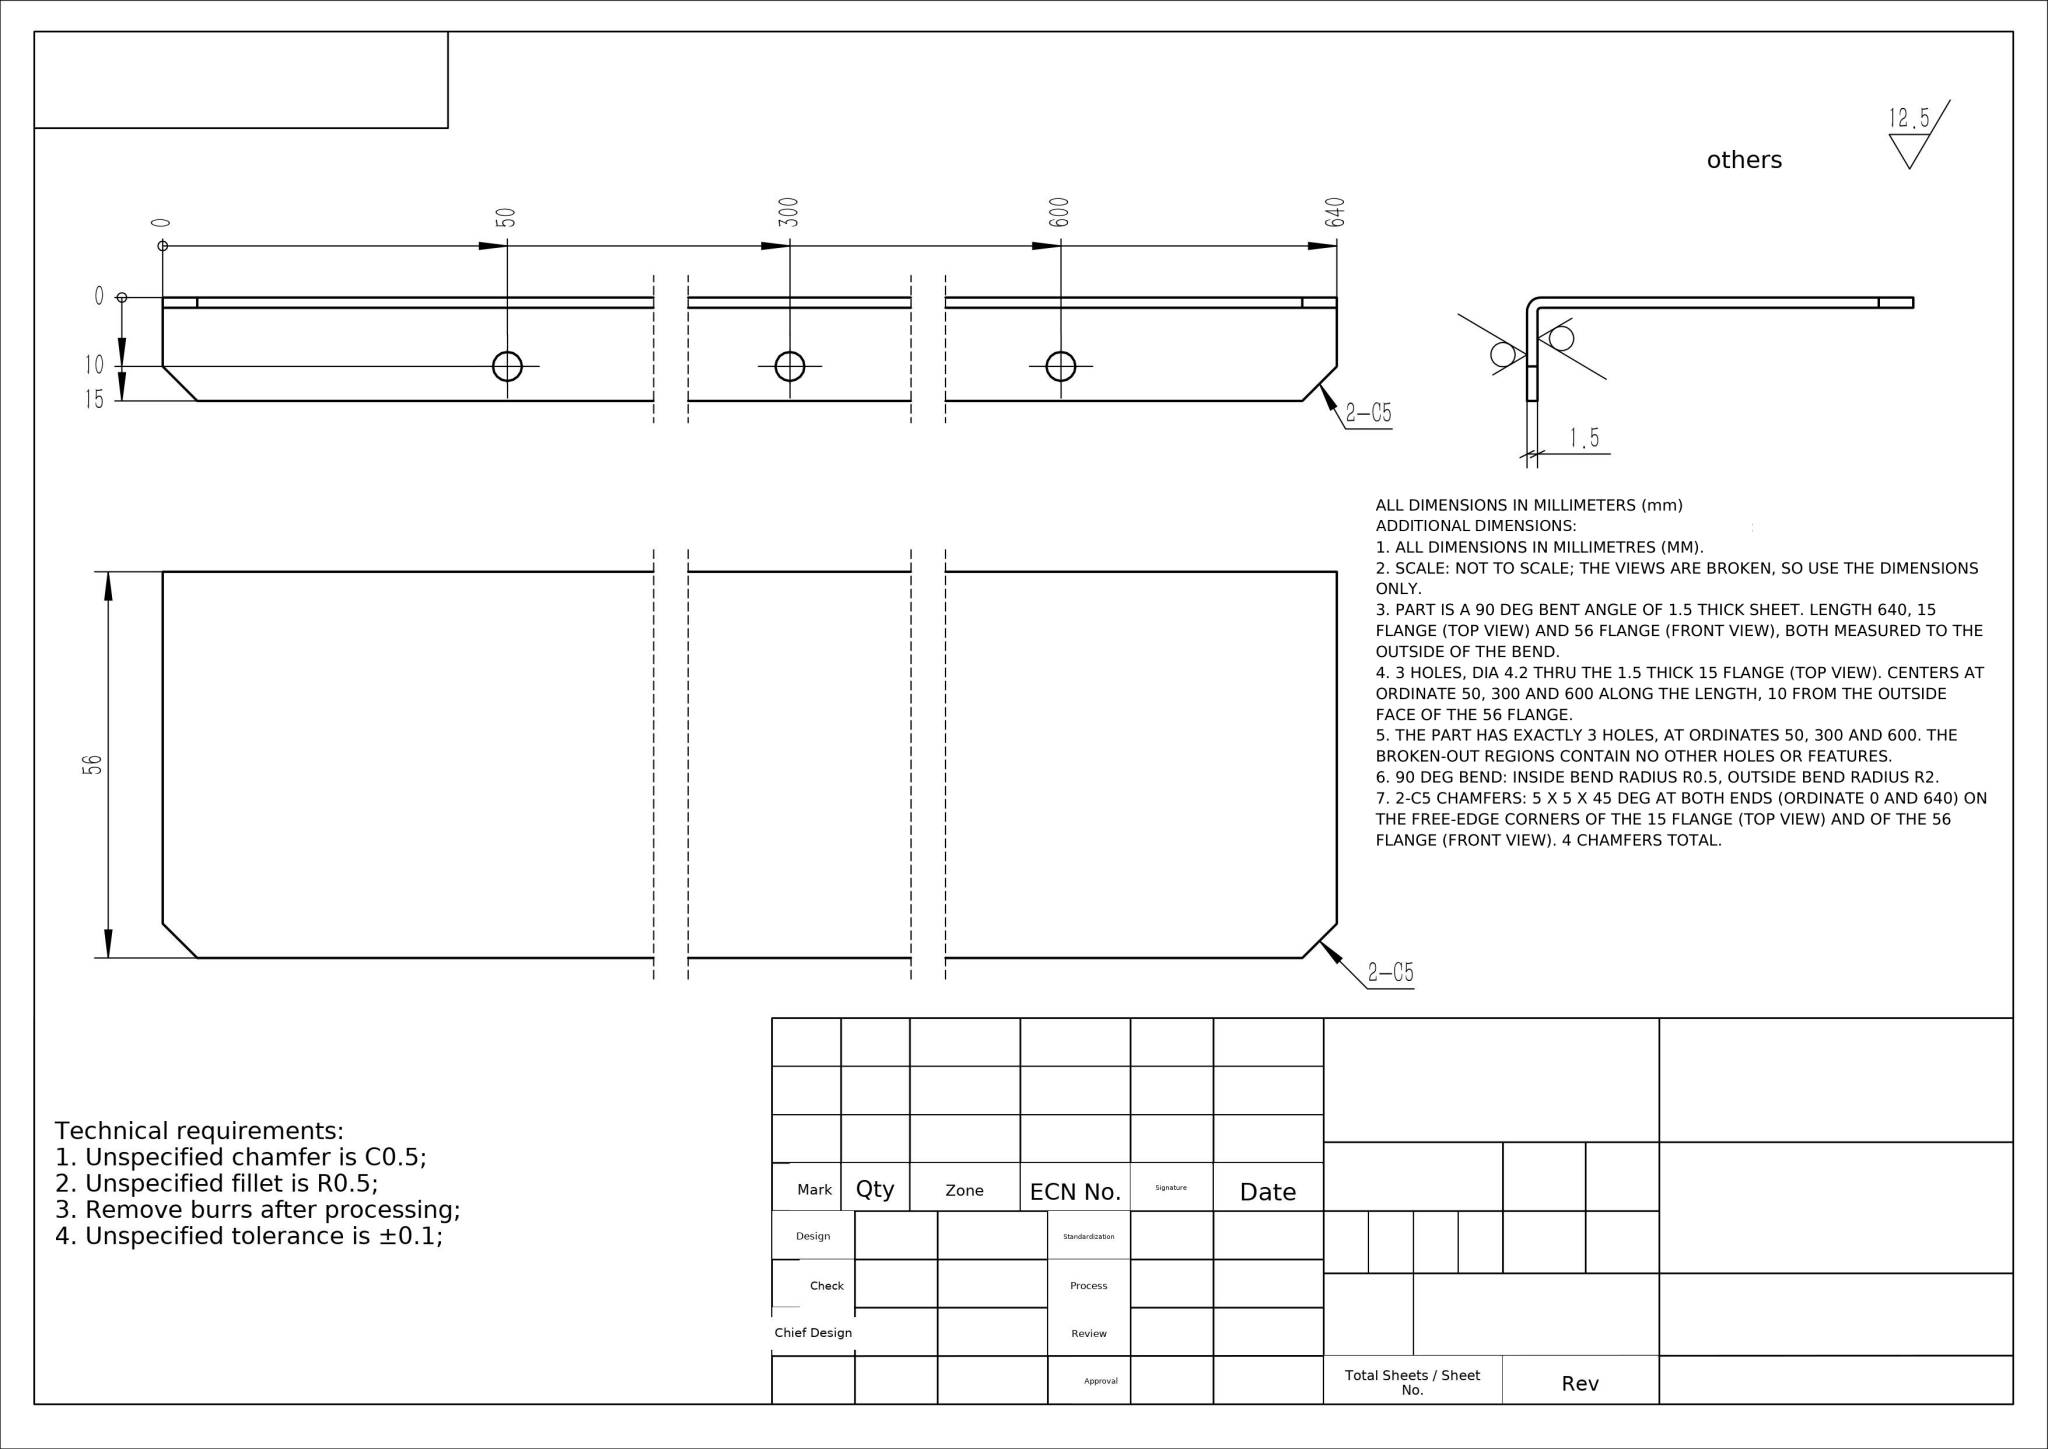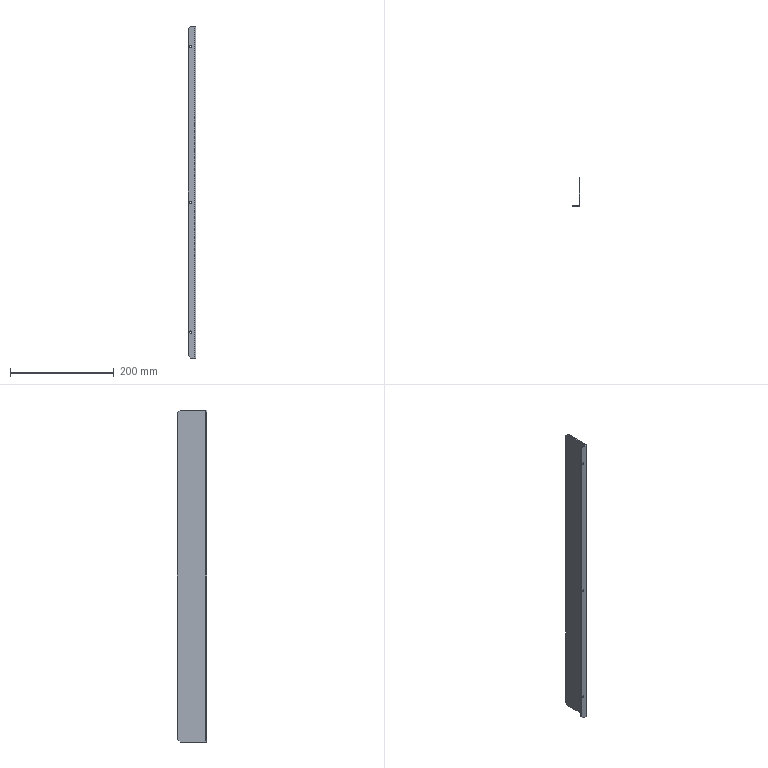Part | NX | mm | 403 | 1 solid | 24 faces | box 15 x 56 x 640 mm | volume 66068 mm3 | plane 16 | cylinder 8 | commonest cylinder face diameters 4.2 x6 1 x1 4 x1
STEP:
#1=COLOUR_RGB('',0.7765,0.7569,0.7373);
#2=FILL_AREA_STYLE_COLOUR('',#1);
#3=FILL_AREA_STYLE('',(#2));
#4=SURFACE_STYLE_FILL_AREA(#3);
#5=SURFACE_SIDE_STYLE('',(#4));
#6=SURFACE_STYLE_USAGE(.BOTH.,#5);
#7=PRESENTATION_STYLE_ASSIGNMENT((#6));
#8=CARTESIAN_POINT('',(-10.,0.,297.9));
#9=VERTEX_POINT('',#8);
#10=CARTESIAN_POINT('',(-10.,0.,302.1));
#11=VERTEX_POINT('',#10);
#12=CARTESIAN_POINT('',(-10.,0.,300.));
#13=DIRECTION('',(0.,1.,0.));
#14=DIRECTION('',(0.,0.,1.));
#15=AXIS2_PLACEMENT_3D('',#12,#13,#14);
#16=CIRCLE('',#15,2.1);
#17=EDGE_CURVE('',#9,#11,#16,.T.);
#18=ORIENTED_EDGE('',*,*,#17,.F.);
#19=CARTESIAN_POINT('',(-10.,1.5,297.9));
#20=VERTEX_POINT('',#19);
#21=CARTESIAN_POINT('',(-10.,0.,297.9));
#22=DIRECTION('',(0.,1.,0.));
#23=VECTOR('',#22,1000.);
#24=LINE('',#21,#23);
#25=EDGE_CURVE('',#9,#20,#24,.T.);
#26=ORIENTED_EDGE('',*,*,#25,.T.);
#27=CARTESIAN_POINT('',(-10.,1.5,302.1));
#28=VERTEX_POINT('',#27);
#29=CARTESIAN_POINT('',(-10.,1.5,300.));
#30=DIRECTION('',(0.,1.,0.));
#31=DIRECTION('',(0.,0.,1.));
#32=AXIS2_PLACEMENT_3D('',#29,#30,#31);
#33=CIRCLE('',#32,2.1);
#34=EDGE_CURVE('',#20,#28,#33,.T.);
#35=ORIENTED_EDGE('',*,*,#34,.T.);
#36=CARTESIAN_POINT('',(-10.,0.,302.1));
#37=DIRECTION('',(0.,1.,0.));
#38=VECTOR('',#37,1000.);
#39=LINE('',#36,#38);
#40=EDGE_CURVE('',#11,#28,#39,.T.);
#41=ORIENTED_EDGE('',*,*,#40,.F.);
#42=EDGE_LOOP('',(#18,#26,#35,#41));
#43=FACE_OUTER_BOUND('',#42,.T.);
#44=CARTESIAN_POINT('',(-10.,0.,300.));
#45=DIRECTION('',(0.,1.,0.));
#46=DIRECTION('',(0.,0.,1.));
#47=AXIS2_PLACEMENT_3D('',#44,#45,#46);
#48=CYLINDRICAL_SURFACE('',#47,2.1);
#49=ADVANCED_FACE('',(#43),#48,.F.);
#50=CARTESIAN_POINT('',(-10.,0.,597.9));
#51=VERTEX_POINT('',#50);
#52=CARTESIAN_POINT('',(-10.,0.,602.1));
#53=VERTEX_POINT('',#52);
#54=CARTESIAN_POINT('',(-10.,0.,600.));
#55=DIRECTION('',(0.,1.,0.));
#56=DIRECTION('',(0.,0.,-1.));
#57=AXIS2_PLACEMENT_3D('',#54,#55,#56);
#58=CIRCLE('',#57,2.1);
#59=EDGE_CURVE('',#51,#53,#58,.T.);
#60=ORIENTED_EDGE('',*,*,#59,.F.);
#61=CARTESIAN_POINT('',(-10.,1.5,597.9));
#62=VERTEX_POINT('',#61);
#63=CARTESIAN_POINT('',(-10.,0.,597.9));
#64=DIRECTION('',(0.,1.,0.));
#65=VECTOR('',#64,1000.);
#66=LINE('',#63,#65);
#67=EDGE_CURVE('',#51,#62,#66,.T.);
#68=ORIENTED_EDGE('',*,*,#67,.T.);
#69=CARTESIAN_POINT('',(-10.,1.5,602.1));
#70=VERTEX_POINT('',#69);
#71=CARTESIAN_POINT('',(-10.,1.5,600.));
#72=DIRECTION('',(0.,1.,0.));
#73=DIRECTION('',(0.,0.,-1.));
#74=AXIS2_PLACEMENT_3D('',#71,#72,#73);
#75=CIRCLE('',#74,2.1);
#76=EDGE_CURVE('',#62,#70,#75,.T.);
#77=ORIENTED_EDGE('',*,*,#76,.T.);
#78=CARTESIAN_POINT('',(-10.,0.,602.1));
#79=DIRECTION('',(0.,1.,0.));
#80=VECTOR('',#79,1000.);
#81=LINE('',#78,#80);
#82=EDGE_CURVE('',#53,#70,#81,.T.);
#83=ORIENTED_EDGE('',*,*,#82,.F.);
#84=EDGE_LOOP('',(#60,#68,#77,#83));
#85=FACE_OUTER_BOUND('',#84,.T.);
#86=CARTESIAN_POINT('',(-10.,0.,600.));
#87=DIRECTION('',(0.,1.,0.));
#88=DIRECTION('',(0.,0.,1.));
#89=AXIS2_PLACEMENT_3D('',#86,#87,#88);
#90=CYLINDRICAL_SURFACE('',#89,2.1);
#91=ADVANCED_FACE('',(#85),#90,.F.);
#92=CARTESIAN_POINT('',(-10.,0.,47.9));
#93=VERTEX_POINT('',#92);
#94=CARTESIAN_POINT('',(-10.,0.,52.1));
#95=VERTEX_POINT('',#94);
#96=CARTESIAN_POINT('',(-10.,0.,50.));
#97=DIRECTION('',(0.,1.,0.));
#98=DIRECTION('',(0.,0.,1.));
#99=AXIS2_PLACEMENT_3D('',#96,#97,#98);
#100=CIRCLE('',#99,2.1);
#101=EDGE_CURVE('',#93,#95,#100,.T.);
#102=ORIENTED_EDGE('',*,*,#101,.F.);
#103=CARTESIAN_POINT('',(-10.,1.5,47.9));
#104=VERTEX_POINT('',#103);
#105=CARTESIAN_POINT('',(-10.,0.,47.9));
#106=DIRECTION('',(0.,1.,0.));
#107=VECTOR('',#106,1000.);
#108=LINE('',#105,#107);
#109=EDGE_CURVE('',#93,#104,#108,.T.);
#110=ORIENTED_EDGE('',*,*,#109,.T.);
#111=CARTESIAN_POINT('',(-10.,1.5,52.1));
#112=VERTEX_POINT('',#111);
#113=CARTESIAN_POINT('',(-10.,1.5,50.));
#114=DIRECTION('',(0.,1.,0.));
#115=DIRECTION('',(0.,0.,1.));
#116=AXIS2_PLACEMENT_3D('',#113,#114,#115);
#117=CIRCLE('',#116,2.1);
#118=EDGE_CURVE('',#104,#112,#117,.T.);
#119=ORIENTED_EDGE('',*,*,#118,.T.);
#120=CARTESIAN_POINT('',(-10.,0.,52.1));
#121=DIRECTION('',(0.,1.,0.));
#122=VECTOR('',#121,1000.);
#123=LINE('',#120,#122);
#124=EDGE_CURVE('',#95,#112,#123,.T.);
#125=ORIENTED_EDGE('',*,*,#124,.F.);
#126=EDGE_LOOP('',(#102,#110,#119,#125));
#127=FACE_OUTER_BOUND('',#126,.T.);
#128=CARTESIAN_POINT('',(-10.,0.,50.));
#129=DIRECTION('',(0.,1.,0.));
#130=DIRECTION('',(0.,0.,1.));
#131=AXIS2_PLACEMENT_3D('',#128,#129,#130);
#132=CYLINDRICAL_SURFACE('',#131,2.1);
#133=ADVANCED_FACE('',(#127),#132,.F.);
#134=CARTESIAN_POINT('',(-2.,0.,640.));
#135=VERTEX_POINT('',#134);
#136=CARTESIAN_POINT('',(-2.,1.5,640.));
#137=VERTEX_POINT('',#136);
#138=CARTESIAN_POINT('',(-2.,0.,640.));
#139=DIRECTION('',(0.,1.,0.));
#140=VECTOR('',#139,1000.);
#141=LINE('',#138,#140);
#142=EDGE_CURVE('',#135,#137,#141,.T.);
#143=ORIENTED_EDGE('',*,*,#142,.F.);
#144=CARTESIAN_POINT('',(0.,2.,640.));
#145=VERTEX_POINT('',#144);
#146=CARTESIAN_POINT('',(-2.,2.,640.));
#147=DIRECTION('',(0.,0.,1.));
#148=DIRECTION('',(-1.,0.,0.));
#149=AXIS2_PLACEMENT_3D('',#146,#147,#148);
#150=CIRCLE('',#149,2.);
#151=EDGE_CURVE('',#135,#145,#150,.T.);
#152=ORIENTED_EDGE('',*,*,#151,.T.);
#153=CARTESIAN_POINT('',(-1.5,2.,640.));
#154=VERTEX_POINT('',#153);
#155=CARTESIAN_POINT('',(-1.5,2.,640.));
#156=DIRECTION('',(1.,0.,0.));
#157=VECTOR('',#156,1000.);
#158=LINE('',#155,#157);
#159=EDGE_CURVE('',#154,#145,#158,.T.);
#160=ORIENTED_EDGE('',*,*,#159,.F.);
#161=CARTESIAN_POINT('',(-2.,2.,640.));
#162=DIRECTION('',(0.,0.,1.));
#163=DIRECTION('',(1.,0.,0.));
#164=AXIS2_PLACEMENT_3D('',#161,#162,#163);
#165=CIRCLE('',#164,0.5);
#166=EDGE_CURVE('',#137,#154,#165,.T.);
#167=ORIENTED_EDGE('',*,*,#166,.F.);
#168=EDGE_LOOP('',(#143,#152,#160,#167));
#169=FACE_OUTER_BOUND('',#168,.T.);
#170=CARTESIAN_POINT('',(-2.,0.,640.));
#171=DIRECTION('',(0.,0.,1.));
#172=DIRECTION('',(1.,0.,0.));
#173=AXIS2_PLACEMENT_3D('',#170,#171,#172);
#174=PLANE('',#173);
#175=ADVANCED_FACE('',(#169),#174,.T.);
#176=CARTESIAN_POINT('',(-10.,1.5,640.));
#177=VERTEX_POINT('',#176);
#178=CARTESIAN_POINT('',(-15.,1.5,640.));
#179=DIRECTION('',(1.,0.,0.));
#180=VECTOR('',#179,1000.);
#181=LINE('',#178,#180);
#182=EDGE_CURVE('',#177,#137,#181,.T.);
#183=ORIENTED_EDGE('',*,*,#182,.F.);
#184=CARTESIAN_POINT('',(-10.,0.,640.));
#185=VERTEX_POINT('',#184);
#186=CARTESIAN_POINT('',(-10.,2.,640.));
#187=DIRECTION('',(0.,-1.,0.));
#188=VECTOR('',#187,1000.);
#189=LINE('',#186,#188);
#190=EDGE_CURVE('',#177,#185,#189,.T.);
#191=ORIENTED_EDGE('',*,*,#190,.T.);
#192=CARTESIAN_POINT('',(-15.,0.,640.));
#193=DIRECTION('',(1.,0.,0.));
#194=VECTOR('',#193,1000.);
#195=LINE('',#192,#194);
#196=EDGE_CURVE('',#185,#135,#195,.T.);
#197=ORIENTED_EDGE('',*,*,#196,.T.);
#198=ORIENTED_EDGE('',*,*,#142,.T.);
#199=EDGE_LOOP('',(#183,#191,#197,#198));
#200=FACE_OUTER_BOUND('',#199,.T.);
#201=CARTESIAN_POINT('',(-1.5,2.,640.));
#202=DIRECTION('',(0.,0.,1.));
#203=DIRECTION('',(1.,0.,0.));
#204=AXIS2_PLACEMENT_3D('',#201,#202,#203);
#205=PLANE('',#204);
#206=ADVANCED_FACE('',(#200),#205,.T.);
#207=CARTESIAN_POINT('',(0.,2.,0.));
#208=VERTEX_POINT('',#207);
#209=CARTESIAN_POINT('',(-1.5,2.,0.));
#210=VERTEX_POINT('',#209);
#211=CARTESIAN_POINT('',(0.,2.,0.));
#212=DIRECTION('',(-1.,0.,0.));
#213=VECTOR('',#212,1000.);
#214=LINE('',#211,#213);
#215=EDGE_CURVE('',#208,#210,#214,.T.);
#216=ORIENTED_EDGE('',*,*,#215,.F.);
#217=CARTESIAN_POINT('',(-2.,0.,0.));
#218=VERTEX_POINT('',#217);
#219=CARTESIAN_POINT('',(-2.,2.,0.));
#220=DIRECTION('',(0.,0.,1.));
#221=DIRECTION('',(-1.,0.,0.));
#222=AXIS2_PLACEMENT_3D('',#219,#220,#221);
#223=CIRCLE('',#222,2.);
#224=EDGE_CURVE('',#218,#208,#223,.T.);
#225=ORIENTED_EDGE('',*,*,#224,.F.);
#226=CARTESIAN_POINT('',(-2.,1.5,0.));
#227=VERTEX_POINT('',#226);
#228=CARTESIAN_POINT('',(-2.,1.5,0.));
#229=DIRECTION('',(0.,-1.,0.));
#230=VECTOR('',#229,1000.);
#231=LINE('',#228,#230);
#232=EDGE_CURVE('',#227,#218,#231,.T.);
#233=ORIENTED_EDGE('',*,*,#232,.F.);
#234=CARTESIAN_POINT('',(-2.,2.,0.));
#235=DIRECTION('',(0.,0.,1.));
#236=DIRECTION('',(1.,0.,0.));
#237=AXIS2_PLACEMENT_3D('',#234,#235,#236);
#238=CIRCLE('',#237,0.5);
#239=EDGE_CURVE('',#227,#210,#238,.T.);
#240=ORIENTED_EDGE('',*,*,#239,.T.);
#241=EDGE_LOOP('',(#216,#225,#233,#240));
#242=FACE_OUTER_BOUND('',#241,.T.);
#243=CARTESIAN_POINT('',(0.,2.,0.));
#244=DIRECTION('',(0.,0.,-1.));
#245=DIRECTION('',(-1.,0.,0.));
#246=AXIS2_PLACEMENT_3D('',#243,#244,#245);
#247=PLANE('',#246);
#248=ADVANCED_FACE('',(#242),#247,.T.);
#249=CARTESIAN_POINT('',(-1.5,51.,-0.));
#250=VERTEX_POINT('',#249);
#251=CARTESIAN_POINT('',(-1.5,0.,0.));
#252=DIRECTION('',(0.,1.,0.));
#253=VECTOR('',#252,1000.);
#254=LINE('',#251,#253);
#255=EDGE_CURVE('',#210,#250,#254,.T.);
#256=ORIENTED_EDGE('',*,*,#255,.T.);
#257=CARTESIAN_POINT('',(0.,51.,-0.));
#258=VERTEX_POINT('',#257);
#259=CARTESIAN_POINT('',(-2.,51.,0.));
#260=DIRECTION('',(1.,0.,0.));
#261=VECTOR('',#260,1000.);
#262=LINE('',#259,#261);
#263=EDGE_CURVE('',#250,#258,#262,.T.);
#264=ORIENTED_EDGE('',*,*,#263,.T.);
#265=CARTESIAN_POINT('',(0.,0.,0.));
#266=DIRECTION('',(0.,1.,0.));
#267=VECTOR('',#266,1000.);
#268=LINE('',#265,#267);
#269=EDGE_CURVE('',#208,#258,#268,.T.);
#270=ORIENTED_EDGE('',*,*,#269,.F.);
#271=ORIENTED_EDGE('',*,*,#215,.T.);
#272=EDGE_LOOP('',(#256,#264,#270,#271));
#273=FACE_OUTER_BOUND('',#272,.T.);
#274=CARTESIAN_POINT('',(-2.,1.5,0.));
#275=DIRECTION('',(0.,0.,-1.));
#276=DIRECTION('',(-1.,0.,0.));
#277=AXIS2_PLACEMENT_3D('',#274,#275,#276);
#278=PLANE('',#277);
#279=ADVANCED_FACE('',(#273),#278,.T.);
#280=ORIENTED_EDGE('',*,*,#269,.T.);
#281=CARTESIAN_POINT('',(0.,56.,5.));
#282=VERTEX_POINT('',#281);
#283=CARTESIAN_POINT('',(0.,51.,0.));
#284=DIRECTION('',(0.,0.7071,0.7071));
#285=VECTOR('',#284,1000.);
#286=LINE('',#283,#285);
#287=EDGE_CURVE('',#258,#282,#286,.T.);
#288=ORIENTED_EDGE('',*,*,#287,.T.);
#289=CARTESIAN_POINT('',(0.,56.,635.));
#290=VERTEX_POINT('',#289);
#291=CARTESIAN_POINT('',(0.,56.,640.));
#292=DIRECTION('',(0.,0.,-1.));
#293=VECTOR('',#292,1000.);
#294=LINE('',#291,#293);
#295=EDGE_CURVE('',#290,#282,#294,.T.);
#296=ORIENTED_EDGE('',*,*,#295,.F.);
#297=CARTESIAN_POINT('',(0.,51.,640.));
#298=VERTEX_POINT('',#297);
#299=CARTESIAN_POINT('',(0.,56.,635.));
#300=DIRECTION('',(0.,-0.7071,0.7071));
#301=VECTOR('',#300,1000.);
#302=LINE('',#299,#301);
#303=EDGE_CURVE('',#290,#298,#302,.T.);
#304=ORIENTED_EDGE('',*,*,#303,.T.);
#305=CARTESIAN_POINT('',(0.,0.,640.));
#306=DIRECTION('',(0.,1.,0.));
#307=VECTOR('',#306,1000.);
#308=LINE('',#305,#307);
#309=EDGE_CURVE('',#145,#298,#308,.T.);
#310=ORIENTED_EDGE('',*,*,#309,.F.);
#311=CARTESIAN_POINT('',(0.,2.,640.));
#312=DIRECTION('',(0.,0.,-1.));
#313=VECTOR('',#312,1000.);
#314=LINE('',#311,#313);
#315=EDGE_CURVE('',#145,#208,#314,.T.);
#316=ORIENTED_EDGE('',*,*,#315,.T.);
#317=EDGE_LOOP('',(#280,#288,#296,#304,#310,#316));
#318=FACE_OUTER_BOUND('',#317,.T.);
#319=CARTESIAN_POINT('',(0.,0.,640.));
#320=DIRECTION('',(-1.,0.,0.));
#321=DIRECTION('',(0.,0.,1.));
#322=AXIS2_PLACEMENT_3D('',#319,#320,#321);
#323=PLANE('',#322);
#324=ADVANCED_FACE('',(#318),#323,.F.);
#325=ORIENTED_EDGE('',*,*,#295,.T.);
#326=CARTESIAN_POINT('',(-1.5,56.,5.));
#327=VERTEX_POINT('',#326);
#328=CARTESIAN_POINT('',(-1.5,56.,5.));
#329=DIRECTION('',(-1.,0.,0.));
#330=VECTOR('',#329,1000.);
#331=LINE('',#328,#330);
#332=EDGE_CURVE('',#282,#327,#331,.T.);
#333=ORIENTED_EDGE('',*,*,#332,.T.);
#334=CARTESIAN_POINT('',(-1.5,56.,635.));
#335=VERTEX_POINT('',#334);
#336=CARTESIAN_POINT('',(-1.5,56.,640.));
#337=DIRECTION('',(0.,0.,-1.));
#338=VECTOR('',#337,1000.);
#339=LINE('',#336,#338);
#340=EDGE_CURVE('',#335,#327,#339,.T.);
#341=ORIENTED_EDGE('',*,*,#340,.F.);
#342=CARTESIAN_POINT('',(-1.5,56.,635.));
#343=DIRECTION('',(1.,0.,0.));
#344=VECTOR('',#343,1000.);
#345=LINE('',#342,#344);
#346=EDGE_CURVE('',#335,#290,#345,.T.);
#347=ORIENTED_EDGE('',*,*,#346,.T.);
#348=EDGE_LOOP('',(#325,#333,#341,#347));
#349=FACE_OUTER_BOUND('',#348,.T.);
#350=CARTESIAN_POINT('',(-1.5,56.,640.));
#351=DIRECTION('',(0.,1.,0.));
#352=DIRECTION('',(0.,0.,1.));
#353=AXIS2_PLACEMENT_3D('',#350,#351,#352);
#354=PLANE('',#353);
#355=ADVANCED_FACE('',(#349),#354,.T.);
#356=ORIENTED_EDGE('',*,*,#340,.T.);
#357=CARTESIAN_POINT('',(-1.5,345.5,294.5));
#358=DIRECTION('',(0.,-0.7071,-0.7071));
#359=VECTOR('',#358,1000.);
#360=LINE('',#357,#359);
#361=EDGE_CURVE('',#327,#250,#360,.T.);
#362=ORIENTED_EDGE('',*,*,#361,.T.);
#363=ORIENTED_EDGE('',*,*,#255,.F.);
#364=CARTESIAN_POINT('',(-1.5,2.,640.));
#365=DIRECTION('',(0.,0.,-1.));
#366=VECTOR('',#365,1000.);
#367=LINE('',#364,#366);
#368=EDGE_CURVE('',#154,#210,#367,.T.);
#369=ORIENTED_EDGE('',*,*,#368,.F.);
#370=CARTESIAN_POINT('',(-1.5,51.,640.));
#371=VERTEX_POINT('',#370);
#372=CARTESIAN_POINT('',(-1.5,0.,640.));
#373=DIRECTION('',(0.,1.,0.));
#374=VECTOR('',#373,1000.);
#375=LINE('',#372,#374);
#376=EDGE_CURVE('',#154,#371,#375,.T.);
#377=ORIENTED_EDGE('',*,*,#376,.T.);
#378=CARTESIAN_POINT('',(-1.5,25.5,665.5));
#379=DIRECTION('',(0.,0.7071,-0.7071));
#380=VECTOR('',#379,1000.);
#381=LINE('',#378,#380);
#382=EDGE_CURVE('',#371,#335,#381,.T.);
#383=ORIENTED_EDGE('',*,*,#382,.T.);
#384=EDGE_LOOP('',(#356,#362,#363,#369,#377,#383));
#385=FACE_OUTER_BOUND('',#384,.T.);
#386=CARTESIAN_POINT('',(-1.5,0.,640.));
#387=DIRECTION('',(-1.,0.,0.));
#388=DIRECTION('',(0.,0.,1.));
#389=AXIS2_PLACEMENT_3D('',#386,#387,#388);
#390=PLANE('',#389);
#391=ADVANCED_FACE('',(#385),#390,.T.);
#392=ORIENTED_EDGE('',*,*,#239,.F.);
#393=CARTESIAN_POINT('',(-2.,1.5,640.));
#394=DIRECTION('',(0.,0.,-1.));
#395=VECTOR('',#394,1000.);
#396=LINE('',#393,#395);
#397=EDGE_CURVE('',#137,#227,#396,.T.);
#398=ORIENTED_EDGE('',*,*,#397,.F.);
#399=ORIENTED_EDGE('',*,*,#166,.T.);
#400=ORIENTED_EDGE('',*,*,#368,.T.);
#401=EDGE_LOOP('',(#392,#398,#399,#400));
#402=FACE_OUTER_BOUND('',#401,.T.);
#403=CARTESIAN_POINT('',(-2.,2.,640.));
#404=DIRECTION('',(0.,0.,-1.));
#405=DIRECTION('',(-1.,0.,0.));
#406=AXIS2_PLACEMENT_3D('',#403,#404,#405);
#407=CYLINDRICAL_SURFACE('',#406,0.5);
#408=ADVANCED_FACE('',(#402),#407,.F.);
#409=CARTESIAN_POINT('',(-10.,1.5,300.));
#410=DIRECTION('',(0.,1.,0.));
#411=DIRECTION('',(0.,0.,1.));
#412=AXIS2_PLACEMENT_3D('',#409,#410,#411);
#413=CIRCLE('',#412,2.1);
#414=EDGE_CURVE('',#28,#20,#413,.T.);
#415=ORIENTED_EDGE('',*,*,#414,.F.);
#416=ORIENTED_EDGE('',*,*,#34,.F.);
#417=EDGE_LOOP('',(#415,#416));
#418=FACE_BOUND('',#417,.T.);
#419=CARTESIAN_POINT('',(-10.,1.5,600.));
#420=DIRECTION('',(0.,1.,0.));
#421=DIRECTION('',(0.,0.,-1.));
#422=AXIS2_PLACEMENT_3D('',#419,#420,#421);
#423=CIRCLE('',#422,2.1);
#424=EDGE_CURVE('',#70,#62,#423,.T.);
#425=ORIENTED_EDGE('',*,*,#424,.F.);
#426=ORIENTED_EDGE('',*,*,#76,.F.);
#427=EDGE_LOOP('',(#425,#426));
#428=FACE_BOUND('',#427,.T.);
#429=CARTESIAN_POINT('',(-10.,1.5,50.));
#430=DIRECTION('',(0.,1.,0.));
#431=DIRECTION('',(0.,0.,1.));
#432=AXIS2_PLACEMENT_3D('',#429,#430,#431);
#433=CIRCLE('',#432,2.1);
#434=EDGE_CURVE('',#112,#104,#433,.T.);
#435=ORIENTED_EDGE('',*,*,#434,.F.);
#436=ORIENTED_EDGE('',*,*,#118,.F.);
#437=EDGE_LOOP('',(#435,#436));
#438=FACE_BOUND('',#437,.T.);
#439=CARTESIAN_POINT('',(-10.,1.5,-0.));
#440=VERTEX_POINT('',#439);
#441=CARTESIAN_POINT('',(-15.,1.5,0.));
#442=DIRECTION('',(1.,0.,0.));
#443=VECTOR('',#442,1000.);
#444=LINE('',#441,#443);
#445=EDGE_CURVE('',#440,#227,#444,.T.);
#446=ORIENTED_EDGE('',*,*,#445,.F.);
#447=CARTESIAN_POINT('',(-15.,1.5,5.));
#448=VERTEX_POINT('',#447);
#449=CARTESIAN_POINT('',(-332.5,1.5,322.5));
#450=DIRECTION('',(-0.7071,0.,0.7071));
#451=VECTOR('',#450,1000.);
#452=LINE('',#449,#451);
#453=EDGE_CURVE('',#440,#448,#452,.T.);
#454=ORIENTED_EDGE('',*,*,#453,.T.);
#455=CARTESIAN_POINT('',(-15.,1.5,635.));
#456=VERTEX_POINT('',#455);
#457=CARTESIAN_POINT('',(-15.,1.5,640.));
#458=DIRECTION('',(0.,0.,-1.));
#459=VECTOR('',#458,1000.);
#460=LINE('',#457,#459);
#461=EDGE_CURVE('',#456,#448,#460,.T.);
#462=ORIENTED_EDGE('',*,*,#461,.F.);
#463=CARTESIAN_POINT('',(-12.5,1.5,637.5));
#464=DIRECTION('',(0.7071,0.,0.7071));
#465=VECTOR('',#464,1000.);
#466=LINE('',#463,#465);
#467=EDGE_CURVE('',#456,#177,#466,.T.);
#468=ORIENTED_EDGE('',*,*,#467,.T.);
#469=ORIENTED_EDGE('',*,*,#182,.T.);
#470=ORIENTED_EDGE('',*,*,#397,.T.);
#471=EDGE_LOOP('',(#446,#454,#462,#468,#469,#470));
#472=FACE_OUTER_BOUND('',#471,.T.);
#473=CARTESIAN_POINT('',(-15.,1.5,640.));
#474=DIRECTION('',(0.,1.,0.));
#475=DIRECTION('',(0.,0.,1.));
#476=AXIS2_PLACEMENT_3D('',#473,#474,#475);
#477=PLANE('',#476);
#478=ADVANCED_FACE('',(#418,#428,#438,#472),#477,.T.);
#479=ORIENTED_EDGE('',*,*,#461,.T.);
#480=CARTESIAN_POINT('',(-15.,0.,5.));
#481=VERTEX_POINT('',#480);
#482=CARTESIAN_POINT('',(-15.,0.,5.));
#483=DIRECTION('',(0.,-1.,0.));
#484=VECTOR('',#483,1000.);
#485=LINE('',#482,#484);
#486=EDGE_CURVE('',#448,#481,#485,.T.);
#487=ORIENTED_EDGE('',*,*,#486,.T.);
#488=CARTESIAN_POINT('',(-15.,0.,635.));
#489=VERTEX_POINT('',#488);
#490=CARTESIAN_POINT('',(-15.,0.,640.));
#491=DIRECTION('',(0.,0.,-1.));
#492=VECTOR('',#491,1000.);
#493=LINE('',#490,#492);
#494=EDGE_CURVE('',#489,#481,#493,.T.);
#495=ORIENTED_EDGE('',*,*,#494,.F.);
#496=CARTESIAN_POINT('',(-15.,0.,635.));
#497=DIRECTION('',(0.,1.,0.));
#498=VECTOR('',#497,1000.);
#499=LINE('',#496,#498);
#500=EDGE_CURVE('',#489,#456,#499,.T.);
#501=ORIENTED_EDGE('',*,*,#500,.T.);
#502=EDGE_LOOP('',(#479,#487,#495,#501));
#503=FACE_OUTER_BOUND('',#502,.T.);
#504=CARTESIAN_POINT('',(-15.,0.,640.));
#505=DIRECTION('',(-1.,0.,0.));
#506=DIRECTION('',(0.,0.,1.));
#507=AXIS2_PLACEMENT_3D('',#504,#505,#506);
#508=PLANE('',#507);
#509=ADVANCED_FACE('',(#503),#508,.T.);
#510=CARTESIAN_POINT('',(-10.,0.,300.));
#511=DIRECTION('',(0.,1.,0.));
#512=DIRECTION('',(0.,0.,1.));
#513=AXIS2_PLACEMENT_3D('',#510,#511,#512);
#514=CIRCLE('',#513,2.1);
#515=EDGE_CURVE('',#11,#9,#514,.T.);
#516=ORIENTED_EDGE('',*,*,#515,.T.);
#517=ORIENTED_EDGE('',*,*,#17,.T.);
#518=EDGE_LOOP('',(#516,#517));
#519=FACE_BOUND('',#518,.T.);
#520=CARTESIAN_POINT('',(-10.,0.,600.));
#521=DIRECTION('',(0.,1.,0.));
#522=DIRECTION('',(0.,0.,-1.));
#523=AXIS2_PLACEMENT_3D('',#520,#521,#522);
#524=CIRCLE('',#523,2.1);
#525=EDGE_CURVE('',#53,#51,#524,.T.);
#526=ORIENTED_EDGE('',*,*,#525,.T.);
#527=ORIENTED_EDGE('',*,*,#59,.T.);
#528=EDGE_LOOP('',(#526,#527));
#529=FACE_BOUND('',#528,.T.);
#530=CARTESIAN_POINT('',(-10.,0.,50.));
#531=DIRECTION('',(0.,1.,0.));
#532=DIRECTION('',(0.,0.,1.));
#533=AXIS2_PLACEMENT_3D('',#530,#531,#532);
#534=CIRCLE('',#533,2.1);
#535=EDGE_CURVE('',#95,#93,#534,.T.);
#536=ORIENTED_EDGE('',*,*,#535,.T.);
#537=ORIENTED_EDGE('',*,*,#101,.T.);
#538=EDGE_LOOP('',(#536,#537));
#539=FACE_BOUND('',#538,.T.);
#540=ORIENTED_EDGE('',*,*,#494,.T.);
#541=CARTESIAN_POINT('',(-10.,0.,0.));
#542=VERTEX_POINT('',#541);
#543=CARTESIAN_POINT('',(-10.,0.,0.));
#544=DIRECTION('',(0.7071,0.,-0.7071));
#545=VECTOR('',#544,1000.);
#546=LINE('',#543,#545);
#547=EDGE_CURVE('',#481,#542,#546,.T.);
#548=ORIENTED_EDGE('',*,*,#547,.T.);
#549=CARTESIAN_POINT('',(-15.,0.,0.));
#550=DIRECTION('',(1.,0.,0.));
#551=VECTOR('',#550,1000.);
#552=LINE('',#549,#551);
#553=EDGE_CURVE('',#542,#218,#552,.T.);
#554=ORIENTED_EDGE('',*,*,#553,.T.);
#555=CARTESIAN_POINT('',(-2.,0.,640.));
#556=DIRECTION('',(0.,0.,-1.));
#557=VECTOR('',#556,1000.);
#558=LINE('',#555,#557);
#559=EDGE_CURVE('',#135,#218,#558,.T.);
#560=ORIENTED_EDGE('',*,*,#559,.F.);
#561=ORIENTED_EDGE('',*,*,#196,.F.);
#562=CARTESIAN_POINT('',(-15.,0.,635.));
#563=DIRECTION('',(-0.7071,0.,-0.7071));
#564=VECTOR('',#563,1000.);
#565=LINE('',#562,#564);
#566=EDGE_CURVE('',#185,#489,#565,.T.);
#567=ORIENTED_EDGE('',*,*,#566,.T.);
#568=EDGE_LOOP('',(#540,#548,#554,#560,#561,#567));
#569=FACE_OUTER_BOUND('',#568,.T.);
#570=CARTESIAN_POINT('',(-15.,0.,640.));
#571=DIRECTION('',(0.,1.,0.));
#572=DIRECTION('',(0.,0.,1.));
#573=AXIS2_PLACEMENT_3D('',#570,#571,#572);
#574=PLANE('',#573);
#575=ADVANCED_FACE('',(#519,#529,#539,#569),#574,.F.);
#576=ORIENTED_EDGE('',*,*,#224,.T.);
#577=ORIENTED_EDGE('',*,*,#315,.F.);
#578=ORIENTED_EDGE('',*,*,#151,.F.);
#579=ORIENTED_EDGE('',*,*,#559,.T.);
#580=EDGE_LOOP('',(#576,#577,#578,#579));
#581=FACE_OUTER_BOUND('',#580,.T.);
#582=CARTESIAN_POINT('',(-2.,2.,640.));
#583=DIRECTION('',(0.,0.,-1.));
#584=DIRECTION('',(-1.,0.,0.));
#585=AXIS2_PLACEMENT_3D('',#582,#583,#584);
#586=CYLINDRICAL_SURFACE('',#585,2.);
#587=ADVANCED_FACE('',(#581),#586,.T.);
#588=ORIENTED_EDGE('',*,*,#309,.T.);
#589=CARTESIAN_POINT('',(-2.,51.,640.));
#590=DIRECTION('',(-1.,0.,0.));
#591=VECTOR('',#590,1000.);
#592=LINE('',#589,#591);
#593=EDGE_CURVE('',#298,#371,#592,.T.);
#594=ORIENTED_EDGE('',*,*,#593,.T.);
#595=ORIENTED_EDGE('',*,*,#376,.F.);
#596=ORIENTED_EDGE('',*,*,#159,.T.);
#597=EDGE_LOOP('',(#588,#594,#595,#596));
#598=FACE_OUTER_BOUND('',#597,.T.);
#599=CARTESIAN_POINT('',(-2.,2.,640.));
#600=DIRECTION('',(0.,0.,1.));
#601=DIRECTION('',(1.,0.,0.));
#602=AXIS2_PLACEMENT_3D('',#599,#600,#601);
#603=PLANE('',#602);
#604=ADVANCED_FACE('',(#598),#603,.T.);
#605=ORIENTED_EDGE('',*,*,#553,.F.);
#606=CARTESIAN_POINT('',(-10.,1.5,0.));
#607=DIRECTION('',(0.,1.,0.));
#608=VECTOR('',#607,1000.);
#609=LINE('',#606,#608);
#610=EDGE_CURVE('',#542,#440,#609,.T.);
#611=ORIENTED_EDGE('',*,*,#610,.T.);
#612=ORIENTED_EDGE('',*,*,#445,.T.);
#613=ORIENTED_EDGE('',*,*,#232,.T.);
#614=EDGE_LOOP('',(#605,#611,#612,#613));
#615=FACE_OUTER_BOUND('',#614,.T.);
#616=CARTESIAN_POINT('',(-2.,2.,0.));
#617=DIRECTION('',(0.,0.,1.));
#618=DIRECTION('',(1.,0.,0.));
#619=AXIS2_PLACEMENT_3D('',#616,#617,#618);
#620=PLANE('',#619);
#621=ADVANCED_FACE('',(#615),#620,.F.);
#622=ORIENTED_EDGE('',*,*,#109,.F.);
#623=ORIENTED_EDGE('',*,*,#535,.F.);
#624=ORIENTED_EDGE('',*,*,#124,.T.);
#625=ORIENTED_EDGE('',*,*,#434,.T.);
#626=EDGE_LOOP('',(#622,#623,#624,#625));
#627=FACE_OUTER_BOUND('',#626,.T.);
#628=CARTESIAN_POINT('',(-10.,0.,50.));
#629=DIRECTION('',(0.,1.,0.));
#630=DIRECTION('',(0.,0.,1.));
#631=AXIS2_PLACEMENT_3D('',#628,#629,#630);
#632=CYLINDRICAL_SURFACE('',#631,2.1);
#633=ADVANCED_FACE('',(#627),#632,.F.);
#634=ORIENTED_EDGE('',*,*,#67,.F.);
#635=ORIENTED_EDGE('',*,*,#525,.F.);
#636=ORIENTED_EDGE('',*,*,#82,.T.);
#637=ORIENTED_EDGE('',*,*,#424,.T.);
#638=EDGE_LOOP('',(#634,#635,#636,#637));
#639=FACE_OUTER_BOUND('',#638,.T.);
#640=CARTESIAN_POINT('',(-10.,0.,600.));
#641=DIRECTION('',(0.,1.,0.));
#642=DIRECTION('',(0.,0.,1.));
#643=AXIS2_PLACEMENT_3D('',#640,#641,#642);
#644=CYLINDRICAL_SURFACE('',#643,2.1);
#645=ADVANCED_FACE('',(#639),#644,.F.);
#646=ORIENTED_EDGE('',*,*,#25,.F.);
#647=ORIENTED_EDGE('',*,*,#515,.F.);
#648=ORIENTED_EDGE('',*,*,#40,.T.);
#649=ORIENTED_EDGE('',*,*,#414,.T.);
#650=EDGE_LOOP('',(#646,#647,#648,#649));
#651=FACE_OUTER_BOUND('',#650,.T.);
#652=CARTESIAN_POINT('',(-10.,0.,300.));
#653=DIRECTION('',(0.,1.,0.));
#654=DIRECTION('',(0.,0.,1.));
#655=AXIS2_PLACEMENT_3D('',#652,#653,#654);
#656=CYLINDRICAL_SURFACE('',#655,2.1);
#657=ADVANCED_FACE('',(#651),#656,.F.);
#658=ORIENTED_EDGE('',*,*,#361,.F.);
#659=ORIENTED_EDGE('',*,*,#332,.F.);
#660=ORIENTED_EDGE('',*,*,#287,.F.);
#661=ORIENTED_EDGE('',*,*,#263,.F.);
#662=EDGE_LOOP('',(#658,#659,#660,#661));
#663=FACE_OUTER_BOUND('',#662,.T.);
#664=CARTESIAN_POINT('',(-2.,51.,0.));
#665=DIRECTION('',(0.,-0.7071,0.7071));
#666=DIRECTION('',(1.,0.,0.));
#667=AXIS2_PLACEMENT_3D('',#664,#665,#666);
#668=PLANE('',#667);
#669=ADVANCED_FACE('',(#663),#668,.F.);
#670=ORIENTED_EDGE('',*,*,#547,.F.);
#671=ORIENTED_EDGE('',*,*,#486,.F.);
#672=ORIENTED_EDGE('',*,*,#453,.F.);
#673=ORIENTED_EDGE('',*,*,#610,.F.);
#674=EDGE_LOOP('',(#670,#671,#672,#673));
#675=FACE_OUTER_BOUND('',#674,.T.);
#676=CARTESIAN_POINT('',(-10.,2.,0.));
#677=DIRECTION('',(-0.7071,0.,-0.7071));
#678=DIRECTION('',(0.,-1.,0.));
#679=AXIS2_PLACEMENT_3D('',#676,#677,#678);
#680=PLANE('',#679);
#681=ADVANCED_FACE('',(#675),#680,.T.);
#682=ORIENTED_EDGE('',*,*,#382,.F.);
#683=ORIENTED_EDGE('',*,*,#593,.F.);
#684=ORIENTED_EDGE('',*,*,#303,.F.);
#685=ORIENTED_EDGE('',*,*,#346,.F.);
#686=EDGE_LOOP('',(#682,#683,#684,#685));
#687=FACE_OUTER_BOUND('',#686,.T.);
#688=CARTESIAN_POINT('',(-1.5,56.,635.));
#689=DIRECTION('',(0.,-0.7071,-0.7071));
#690=DIRECTION('',(1.,0.,0.));
#691=AXIS2_PLACEMENT_3D('',#688,#689,#690);
#692=PLANE('',#691);
#693=ADVANCED_FACE('',(#687),#692,.F.);
#694=ORIENTED_EDGE('',*,*,#566,.F.);
#695=ORIENTED_EDGE('',*,*,#190,.F.);
#696=ORIENTED_EDGE('',*,*,#467,.F.);
#697=ORIENTED_EDGE('',*,*,#500,.F.);
#698=EDGE_LOOP('',(#694,#695,#696,#697));
#699=FACE_OUTER_BOUND('',#698,.T.);
#700=CARTESIAN_POINT('',(-15.,0.,635.));
#701=DIRECTION('',(0.7071,0.,-0.7071));
#702=DIRECTION('',(0.,1.,0.));
#703=AXIS2_PLACEMENT_3D('',#700,#701,#702);
#704=PLANE('',#703);
#705=ADVANCED_FACE('',(#699),#704,.F.);
#706=CLOSED_SHELL('',(#49,#91,#133,#175,#206,#248,#279,#324,#355,#391,#408,#478,#509,#575,#587,#604,#621,#633,#645,#657,#669,#681,#693,#705));
#707=MANIFOLD_SOLID_BREP('',#706);
#708=CARTESIAN_POINT('',(0.,0.,0.));
#709=DIRECTION('',(0.,0.,1.));
#710=DIRECTION('',(1.,0.,0.));
#711=AXIS2_PLACEMENT_3D('',#708,#709,#710);
#712=(LENGTH_UNIT()NAMED_UNIT(*)SI_UNIT(.MILLI.,.METRE.));
#713=UNCERTAINTY_MEASURE_WITH_UNIT(LENGTH_MEASURE(0.00001),#712,'','');
#714=(NAMED_UNIT(*)PLANE_ANGLE_UNIT()SI_UNIT($,.RADIAN.));
#715=(NAMED_UNIT(*)SI_UNIT($,.STERADIAN.)SOLID_ANGLE_UNIT());
#716=(GEOMETRIC_REPRESENTATION_CONTEXT(3)GLOBAL_UNCERTAINTY_ASSIGNED_CONTEXT((#713))GLOBAL_UNIT_ASSIGNED_CONTEXT((#712,#714,#715))REPRESENTATION_CONTEXT('',''));
#717=ADVANCED_BREP_SHAPE_REPRESENTATION('',(#707,#711),#716);
#718=STYLED_ITEM('',(#7),#717);
#719=(LENGTH_UNIT()NAMED_UNIT(*)SI_UNIT(.MILLI.,.METRE.));
#720=UNCERTAINTY_MEASURE_WITH_UNIT(LENGTH_MEASURE(0.00001),#719,'','');
#721=(NAMED_UNIT(*)PLANE_ANGLE_UNIT()SI_UNIT($,.RADIAN.));
#722=(NAMED_UNIT(*)SI_UNIT($,.STERADIAN.)SOLID_ANGLE_UNIT());
#723=(GEOMETRIC_REPRESENTATION_CONTEXT(3)GLOBAL_UNCERTAINTY_ASSIGNED_CONTEXT((#720))GLOBAL_UNIT_ASSIGNED_CONTEXT((#719,#721,#722))REPRESENTATION_CONTEXT('',''));
#724=MECHANICAL_DESIGN_GEOMETRIC_PRESENTATION_REPRESENTATION('',(#718),#723);
#725=COLOUR_RGB('',0.7765,0.7569,0.7373);
#726=FILL_AREA_STYLE_COLOUR('',#725);
#727=FILL_AREA_STYLE('',(#726));
#728=SURFACE_STYLE_FILL_AREA(#727);
#729=SURFACE_SIDE_STYLE('',(#728));
#730=SURFACE_STYLE_USAGE(.BOTH.,#729);
#731=PRESENTATION_STYLE_ASSIGNMENT((#730));
#732=STYLED_ITEM('',(#731),#707);
#733=(LENGTH_UNIT()NAMED_UNIT(*)SI_UNIT(.MILLI.,.METRE.));
#734=UNCERTAINTY_MEASURE_WITH_UNIT(LENGTH_MEASURE(0.00001),#733,'','');
#735=(NAMED_UNIT(*)PLANE_ANGLE_UNIT()SI_UNIT($,.RADIAN.));
#736=(NAMED_UNIT(*)SI_UNIT($,.STERADIAN.)SOLID_ANGLE_UNIT());
#737=(GEOMETRIC_REPRESENTATION_CONTEXT(3)GLOBAL_UNCERTAINTY_ASSIGNED_CONTEXT((#734))GLOBAL_UNIT_ASSIGNED_CONTEXT((#733,#735,#736))REPRESENTATION_CONTEXT('',''));
#738=MECHANICAL_DESIGN_GEOMETRIC_PRESENTATION_REPRESENTATION('',(#732),#737);
#739=PRESENTATION_LAYER_ASSIGNMENT('','',(#732));
#740=PRESENTATION_LAYER_ASSIGNMENT('','',(#718));